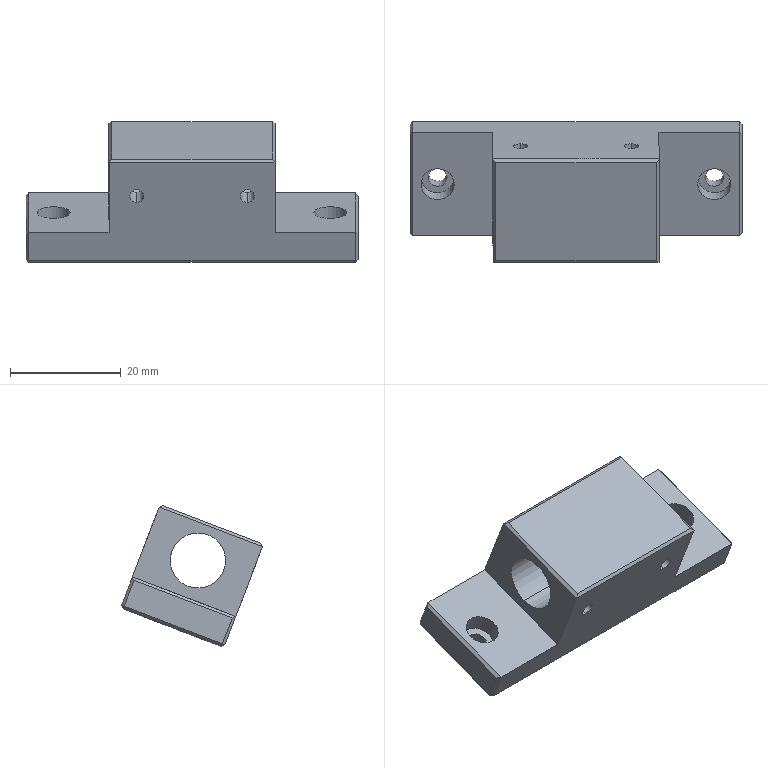Component | SolidWorks | XM-WST05-2003-1 | 1 solid | 48 faces | box 60 x 25.47 x 25.47 mm | volume 12866 mm3 | plane 30 | cylinder 18 | commonest cylinder face diameters 2.5 x8 6 x4 3.4 x4 10 x2
build123d program:
from build123d import *

# Parameters (mm, degrees)
SKETCH2_W                                            = 60
SKETCH2_H                                            = 20
BOSS_EXTRUDE1_DEPTH                                  = 20
SKETCH3_W                                            = 15
SKETCH3_H                                            = 14
CUT_EXTRUDE1_DEPTH                                   = 42.231
SKETCH4_R                                            = 5
CUT_EXTRUDE3_DEPTH                                   = 51.249
HOLE_SIZE_ACCORDING_TO_THE_TYPE_OF_HEX_S_D           = 3.4
HOLE_SIZE_ACCORDING_TO_THE_TYPE_OF_HEX_S_CBORE_D     = 6
HOLE_SIZE_ACCORDING_TO_THE_TYPE_OF_HEX_S_CBORE_DEPTH = 3.4
M3_TAPPED_HOLE1_D                                    = 2.5
CHAMFER1_SIZE                                        = 0.5


with BuildPart() as part:
    # Sketch2 → Boss-Extrude1 (new body)
    with BuildSketch(Plane.XY):
        Rectangle(SKETCH2_W, SKETCH2_H)
    extrude(amount=BOSS_EXTRUDE1_DEPTH)

    # Sketch3 → Cut-Extrude1 (cut, through all)
    with BuildSketch(Plane(origin=(0, 10, 0), x_dir=(1, 0, 0), z_dir=(0, 1, 0))):
        with Locations((-22.5, -13)):
            Rectangle(SKETCH3_W, SKETCH3_H)
        with Locations((22.5, -13)):
            Rectangle(SKETCH3_W, SKETCH3_H)
    extrude(amount=-CUT_EXTRUDE1_DEPTH, mode=Mode.SUBTRACT)

    # Sketch4 → Cut-Extrude3 (cut, through all)
    with BuildSketch(Plane(origin=(15, 0, 0), x_dir=(0, 0, -1), z_dir=(1, 0, 0))):
        with Locations((-13, 0)):
            Circle(SKETCH4_R)
    extrude(amount=-CUT_EXTRUDE3_DEPTH, mode=Mode.SUBTRACT)

    # Hole Size according to the type of Hex S (through all)
    with Locations(Plane.XY.offset(6)):
        with Locations((-25, 0), (25, 0)):
            CounterBoreHole(HOLE_SIZE_ACCORDING_TO_THE_TYPE_OF_HEX_S_D / 2, HOLE_SIZE_ACCORDING_TO_THE_TYPE_OF_HEX_S_CBORE_D / 2, HOLE_SIZE_ACCORDING_TO_THE_TYPE_OF_HEX_S_CBORE_DEPTH)

    # M3 Tapped Hole1 (through all)
    with Locations(Plane(origin=(0, 10, 0), x_dir=(1, 0, 0), z_dir=(0, 1, 0))):
        with Locations((-10, -13), (10, -13)):
            Hole(M3_TAPPED_HOLE1_D / 2)

    # Chamfer1
    chamfer1_edges = [part.edges().sort_by_distance(p)[0] for p in [
        (0, -10, 20),
        (-30, -10, 3),
        (-30, 10, 3),
        (-30, 0, 6),
        (-15, 0, 20),
        (0, 10, 20),
        (30, -10, 3),
        (30, 10, 3),
        (30, 0, 6),
        (15, 0, 20),
        (0, -10, 0),
        (-30, 0, 0),
        (0, 10, 0),
        (30, 0, 0),
    ]]
    chamfer(chamfer1_edges, length=CHAMFER1_SIZE)


solid = part.part

# Placed as in the assembly
solid = solid.moved(Location((-143.297, 122.354, 409.108), (20.935, 0, 0)))